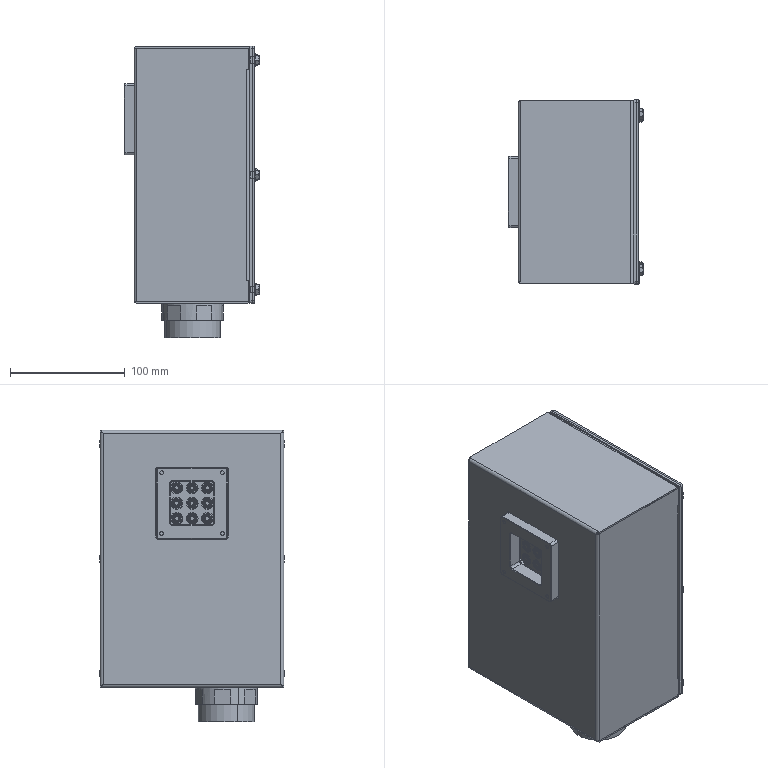CAM job | Mastercam | mm | 15 operations | part box 118.13 x 161 x 254
1. Facing | 24 - 100 平铣刀
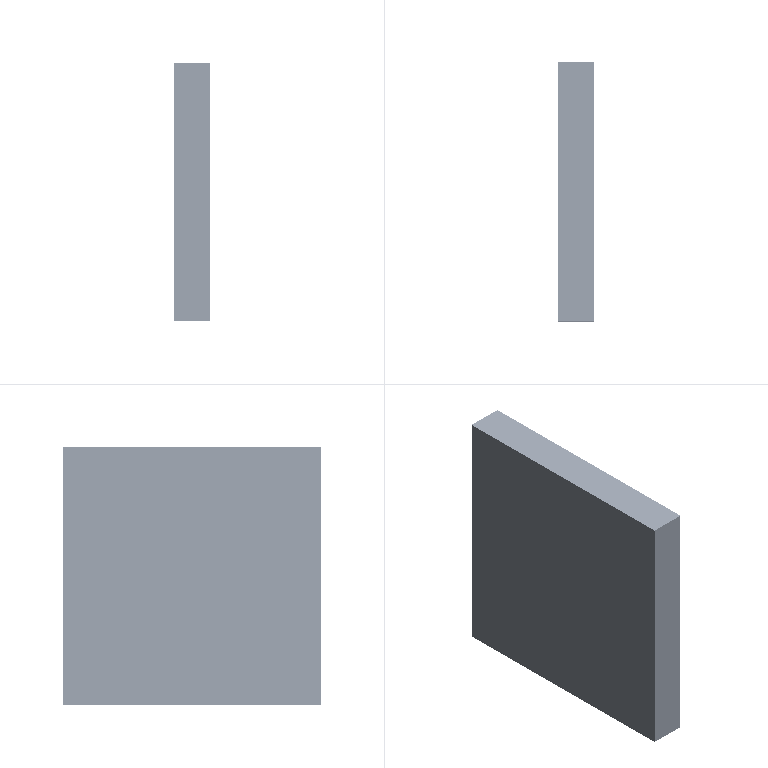2. 3D High Speed (Dynamic OptiRough) | 12 - 12 平铣刀
3. Contour (Ramp) | 14 - 20 平铣刀
4. Facing | 10 - 10 平铣刀
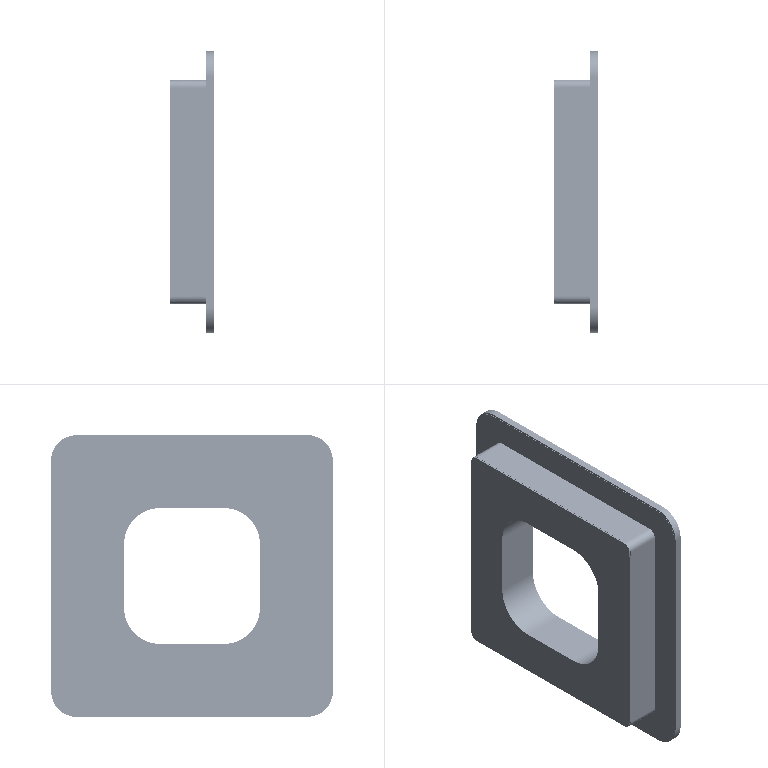5. Contour (Remachining) | 10 - 10 平铣刀
6. Contour (2D) | 10 - 10 平铣刀
7. Contour (2D) | 10 - 10 平铣刀
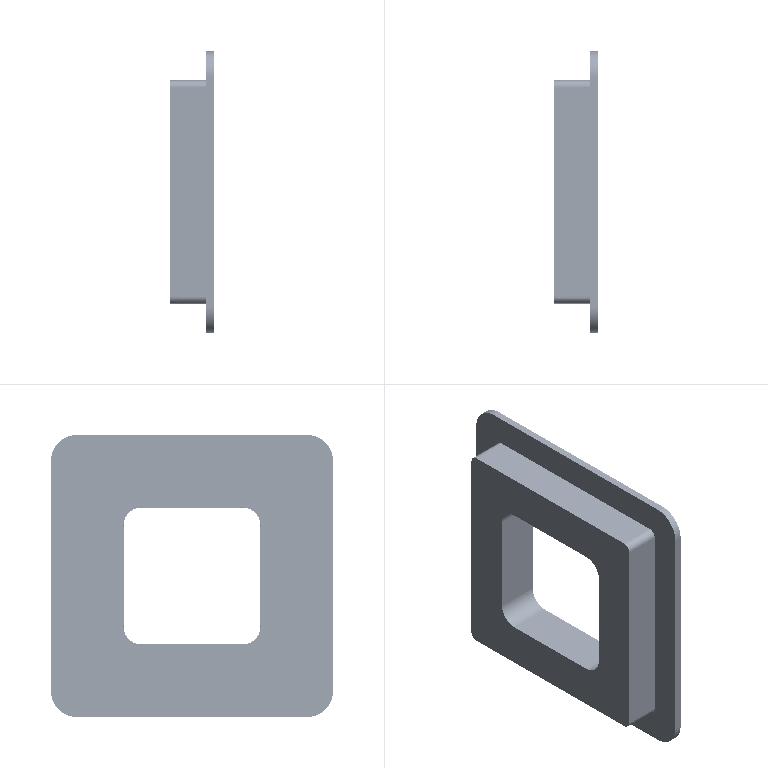8. Contour (2D) | 10 - 10 平铣刀
9. Contour (Remachining) | 4 - 4 平铣刀
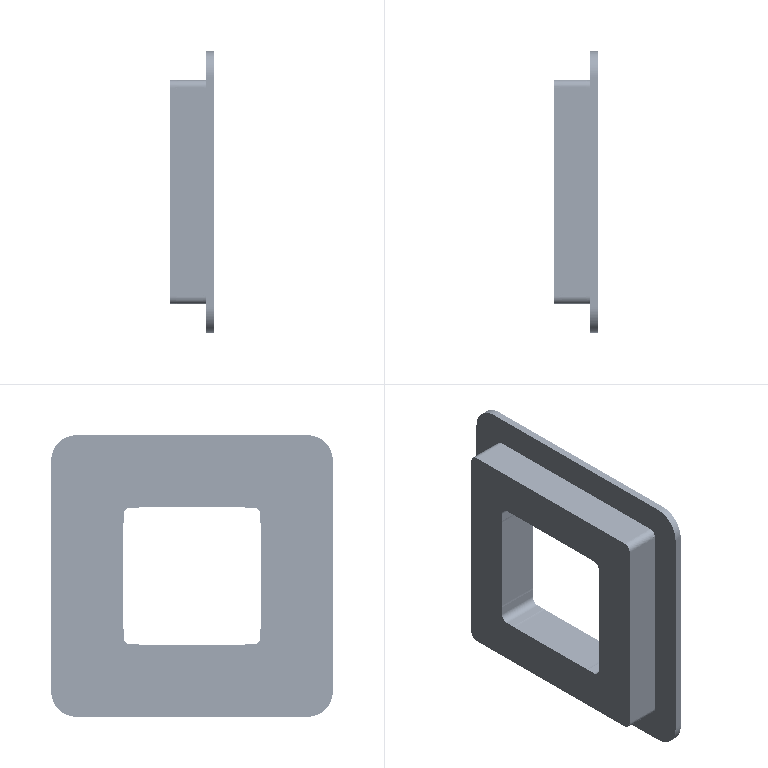10. Contour (Remachining) | 4 - 4 平铣刀
11. Drill/Counterbore | 7 - 10 倒角刀
12. Contour (2D chamfer) | 7 - 10 倒角刀
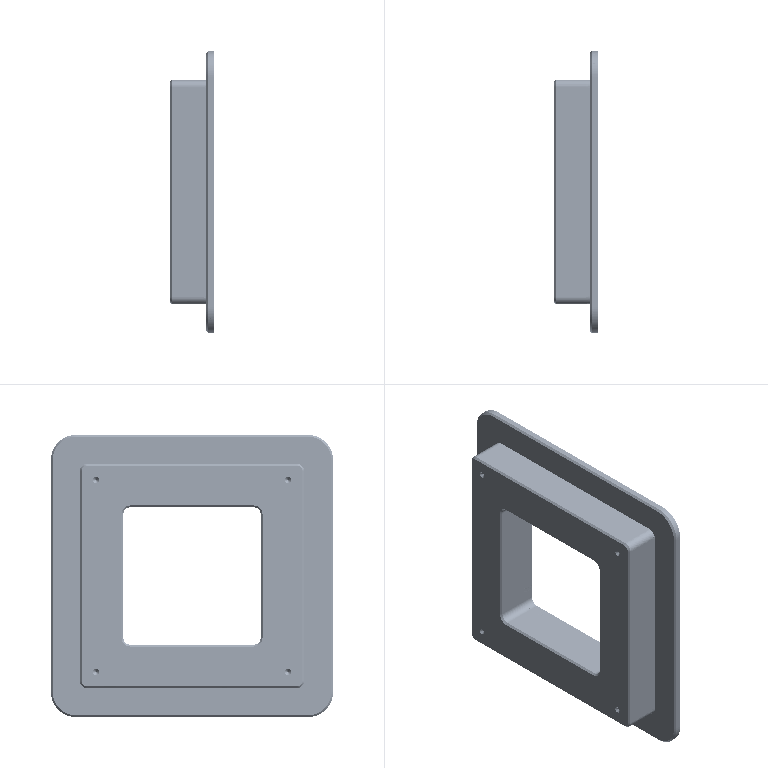13. Facing | 23 - 50 平铣刀
14. Facing | 24 - 100 平铣刀
15. Contour (2D chamfer) | 7 - 10 倒角刀